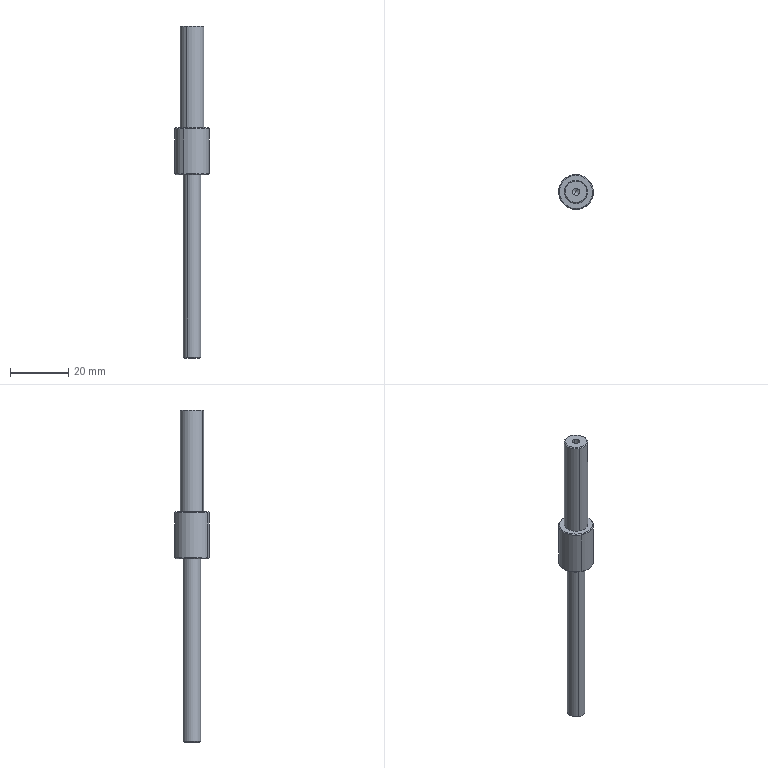Component | SolidWorks | DZ.KX.203-TC1505-20-18-05-96-1 | 1 solid | 26 faces | box 12 x 12 x 114 mm | volume 5230 mm3 | cone 12 | cylinder 10 | plane 4 | commonest cylinder face diameters 2.5 x4 6 x2 12 x2 8 x2 | material Plain Carbon Steel
build123d program:
from build123d import *

# Parameters (mm, degrees)
M3_TAPPED_HOLE1_D     = 2.5
M3_TAPPED_HOLE1_DEPTH = 12.5
M3_TAPPED_HOLE1_TIP   = 0.7511
CHAMFER1_SIZE         = 0.3
M3_TAPPED_HOLE2_D     = 2.5
M3_TAPPED_HOLE2_DEPTH = 10.5
M3_TAPPED_HOLE2_TIP   = 0.7511


with BuildPart() as part:
    # Sketch1 → Revolve1 (revolve)
    with BuildSketch(Plane(origin=(0, 0, 0), x_dir=(0, 0, -1), z_dir=(1, 0, 0))):
        Polygon((0, 0), (0, 114), (4, 114), (4, 79), (6, 79), (6, 63), (3, 63), (3, 0), align=None)
    revolve(axis=Axis((0, 0, 0), (0, 1, 0)))

    # M3 Tapped Hole1
    with Locations(Plane(origin=(0, 114, 0), x_dir=(1, 0, 0), z_dir=(0, 1, 0))):
        with Locations((0, 0)):
            Hole(M3_TAPPED_HOLE1_D / 2, depth=M3_TAPPED_HOLE1_DEPTH)
            with Locations((0, 0, -(M3_TAPPED_HOLE1_DEPTH + M3_TAPPED_HOLE1_TIP / 2))):  # 118° drill point
                Cone(0, M3_TAPPED_HOLE1_D / 2, M3_TAPPED_HOLE1_TIP, mode=Mode.SUBTRACT)

    # Chamfer1
    chamfer1_edges = [part.edges().sort_by_distance(p)[0] for p in [
        (0, 0, 3),
        (0, 63, 6),
        (0, 79, 6),
        (0, 114, 4),
    ]]
    chamfer(chamfer1_edges, length=CHAMFER1_SIZE)

    # M3 Tapped Hole2
    with Locations(Plane(origin=(0, 0, 0), x_dir=(-1, 0, 0), z_dir=(0, -1, 0))):
        with Locations((0, 0)):
            Hole(M3_TAPPED_HOLE2_D / 2, depth=M3_TAPPED_HOLE2_DEPTH)
            with Locations((0, 0, -(M3_TAPPED_HOLE2_DEPTH + M3_TAPPED_HOLE2_TIP / 2))):  # 118° drill point
                Cone(0, M3_TAPPED_HOLE2_D / 2, M3_TAPPED_HOLE2_TIP, mode=Mode.SUBTRACT)


solid = part.part

# Placed as in the assembly
solid = solid.moved(Location((295.5, -817.807, 24.06), (90, 0, 0)))
STEP:
#1=COLOUR_RGB('',0.7922,0.8196,0.9333);
#2=FILL_AREA_STYLE_COLOUR('',#1);
#3=FILL_AREA_STYLE('',(#2));
#4=SURFACE_STYLE_FILL_AREA(#3);
#5=SURFACE_SIDE_STYLE('',(#4));
#6=SURFACE_STYLE_USAGE(.BOTH.,#5);
#7=PRESENTATION_STYLE_ASSIGNMENT((#6));
#8=CARTESIAN_POINT('',(11.61,-32.24,1.361));
#9=VERTEX_POINT('',#8);
#10=CARTESIAN_POINT('',(11.657,-32.154,1.361));
#11=VERTEX_POINT('',#10);
#12=CARTESIAN_POINT('',(11.634,-32.197,1.361));
#13=DIRECTION('',(0.,-0.,-1.));
#14=DIRECTION('',(0.4749,0.88,0.));
#15=AXIS2_PLACEMENT_3D('',#12,#13,#14);
#16=CIRCLE('',#15,0.04921);
#17=EDGE_CURVE('',#9,#11,#16,.T.);
#18=ORIENTED_EDGE('',*,*,#17,.F.);
#19=CARTESIAN_POINT('',(11.61,-32.24,0.9472));
#20=VERTEX_POINT('',#19);
#21=CARTESIAN_POINT('',(11.61,-32.24,0.9472));
#22=DIRECTION('',(0.,-0.,-1.));
#23=VECTOR('',#22,39.37);
#24=LINE('',#21,#23);
#25=EDGE_CURVE('',#9,#20,#24,.T.);
#26=ORIENTED_EDGE('',*,*,#25,.T.);
#27=CARTESIAN_POINT('',(11.657,-32.154,0.9472));
#28=VERTEX_POINT('',#27);
#29=CARTESIAN_POINT('',(11.634,-32.197,0.9472));
#30=DIRECTION('',(0.,-0.,-1.));
#31=DIRECTION('',(0.4749,0.88,-0.));
#32=AXIS2_PLACEMENT_3D('',#29,#30,#31);
#33=CIRCLE('',#32,0.04921);
#34=EDGE_CURVE('',#20,#28,#33,.T.);
#35=ORIENTED_EDGE('',*,*,#34,.T.);
#36=CARTESIAN_POINT('',(11.657,-32.154,0.9472));
#37=DIRECTION('',(0.,-0.,-1.));
#38=VECTOR('',#37,39.37);
#39=LINE('',#36,#38);
#40=EDGE_CURVE('',#11,#28,#39,.T.);
#41=ORIENTED_EDGE('',*,*,#40,.F.);
#42=EDGE_LOOP('',(#18,#26,#35,#41));
#43=FACE_OUTER_BOUND('',#42,.T.);
#44=CARTESIAN_POINT('',(11.634,-32.197,0.9472));
#45=DIRECTION('',(0.,-0.,-1.));
#46=DIRECTION('',(0.4749,0.88,-0.));
#47=AXIS2_PLACEMENT_3D('',#44,#45,#46);
#48=CYLINDRICAL_SURFACE('',#47,0.04921);
#49=ADVANCED_FACE('',(#43),#48,.F.);
#50=CARTESIAN_POINT('',(11.634,-32.197,1.39));
#51=VERTEX_POINT('',#50);
#52=CARTESIAN_POINT('',(11.657,-32.154,1.361));
#53=DIRECTION('',(0.4071,0.7543,-0.515));
#54=VECTOR('',#53,39.37);
#55=LINE('',#52,#54);
#56=EDGE_CURVE('',#51,#11,#55,.T.);
#57=ORIENTED_EDGE('',*,*,#56,.F.);
#58=CARTESIAN_POINT('',(11.61,-32.24,1.361));
#59=DIRECTION('',(-0.4071,-0.7543,-0.515));
#60=VECTOR('',#59,39.37);
#61=LINE('',#58,#60);
#62=EDGE_CURVE('',#51,#9,#61,.T.);
#63=ORIENTED_EDGE('',*,*,#62,.T.);
#64=ORIENTED_EDGE('',*,*,#17,.T.);
#65=EDGE_LOOP('',(#57,#63,#64));
#66=FACE_OUTER_BOUND('',#65,.T.);
#67=CARTESIAN_POINT('',(11.634,-32.197,1.361));
#68=DIRECTION('',(0.,-0.,-1.));
#69=DIRECTION('',(0.4749,0.88,0.));
#70=AXIS2_PLACEMENT_3D('',#67,#68,#69);
#71=CONICAL_SURFACE('',#70,0.04921,1.03);
#72=ADVANCED_FACE('',(#66),#71,.F.);
#73=CARTESIAN_POINT('',(11.565,-32.325,5.435));
#74=VERTEX_POINT('',#73);
#75=CARTESIAN_POINT('',(11.703,-32.069,5.435));
#76=VERTEX_POINT('',#75);
#77=CARTESIAN_POINT('',(11.634,-32.197,5.435));
#78=DIRECTION('',(-0.,0.,1.));
#79=DIRECTION('',(-0.4749,-0.88,0.));
#80=AXIS2_PLACEMENT_3D('',#77,#78,#79);
#81=CIRCLE('',#80,0.1457);
#82=EDGE_CURVE('',#74,#76,#81,.T.);
#83=ORIENTED_EDGE('',*,*,#82,.F.);
#84=CARTESIAN_POINT('',(11.559,-32.336,5.424));
#85=VERTEX_POINT('',#84);
#86=CARTESIAN_POINT('',(11.559,-32.336,5.424));
#87=DIRECTION('',(-0.3358,-0.6223,-0.7071));
#88=VECTOR('',#87,39.37);
#89=LINE('',#86,#88);
#90=EDGE_CURVE('',#74,#85,#89,.T.);
#91=ORIENTED_EDGE('',*,*,#90,.T.);
#92=CARTESIAN_POINT('',(11.709,-32.059,5.424));
#93=VERTEX_POINT('',#92);
#94=CARTESIAN_POINT('',(11.634,-32.197,5.424));
#95=DIRECTION('',(0.,-0.,-1.));
#96=DIRECTION('',(-0.4749,-0.88,0.));
#97=AXIS2_PLACEMENT_3D('',#94,#95,#96);
#98=CIRCLE('',#97,0.1575);
#99=EDGE_CURVE('',#93,#85,#98,.T.);
#100=ORIENTED_EDGE('',*,*,#99,.F.);
#101=CARTESIAN_POINT('',(11.709,-32.059,5.424));
#102=DIRECTION('',(0.3358,0.6223,-0.7071));
#103=VECTOR('',#102,39.37);
#104=LINE('',#101,#103);
#105=EDGE_CURVE('',#76,#93,#104,.T.);
#106=ORIENTED_EDGE('',*,*,#105,.F.);
#107=EDGE_LOOP('',(#83,#91,#100,#106));
#108=FACE_OUTER_BOUND('',#107,.T.);
#109=CARTESIAN_POINT('',(11.634,-32.197,5.424));
#110=DIRECTION('',(0.,-0.,-1.));
#111=DIRECTION('',(0.4749,0.88,0.));
#112=AXIS2_PLACEMENT_3D('',#109,#110,#111);
#113=CONICAL_SURFACE('',#112,0.1575,0.7854);
#114=ADVANCED_FACE('',(#108),#113,.T.);
#115=CARTESIAN_POINT('',(11.684,-32.104,0.9472));
#116=VERTEX_POINT('',#115);
#117=CARTESIAN_POINT('',(11.583,-32.291,0.9472));
#118=VERTEX_POINT('',#117);
#119=CARTESIAN_POINT('',(11.634,-32.197,0.9472));
#120=DIRECTION('',(0.,-0.,-1.));
#121=DIRECTION('',(0.4749,0.88,-0.));
#122=AXIS2_PLACEMENT_3D('',#119,#120,#121);
#123=CIRCLE('',#122,0.1063);
#124=EDGE_CURVE('',#116,#118,#123,.T.);
#125=ORIENTED_EDGE('',*,*,#124,.F.);
#126=CARTESIAN_POINT('',(11.69,-32.093,0.959));
#127=VERTEX_POINT('',#126);
#128=CARTESIAN_POINT('',(11.684,-32.104,0.9472));
#129=DIRECTION('',(0.3358,0.6223,0.7071));
#130=VECTOR('',#129,39.37);
#131=LINE('',#128,#130);
#132=EDGE_CURVE('',#116,#127,#131,.T.);
#133=ORIENTED_EDGE('',*,*,#132,.T.);
#134=CARTESIAN_POINT('',(11.578,-32.301,0.959));
#135=VERTEX_POINT('',#134);
#136=CARTESIAN_POINT('',(11.634,-32.197,0.959));
#137=DIRECTION('',(-0.,0.,1.));
#138=DIRECTION('',(0.4749,0.88,-0.));
#139=AXIS2_PLACEMENT_3D('',#136,#137,#138);
#140=CIRCLE('',#139,0.1181);
#141=EDGE_CURVE('',#135,#127,#140,.T.);
#142=ORIENTED_EDGE('',*,*,#141,.F.);
#143=CARTESIAN_POINT('',(11.583,-32.291,0.9472));
#144=DIRECTION('',(-0.3358,-0.6223,0.7071));
#145=VECTOR('',#144,39.37);
#146=LINE('',#143,#145);
#147=EDGE_CURVE('',#118,#135,#146,.T.);
#148=ORIENTED_EDGE('',*,*,#147,.F.);
#149=EDGE_LOOP('',(#125,#133,#142,#148));
#150=FACE_OUTER_BOUND('',#149,.T.);
#151=CARTESIAN_POINT('',(11.634,-32.197,0.9472));
#152=DIRECTION('',(-0.,0.,1.));
#153=DIRECTION('',(-0.4749,-0.88,0.));
#154=AXIS2_PLACEMENT_3D('',#151,#152,#153);
#155=CONICAL_SURFACE('',#154,0.1063,0.7854);
#156=ADVANCED_FACE('',(#150),#155,.T.);
#157=CARTESIAN_POINT('',(11.527,-32.395,4.057));
#158=VERTEX_POINT('',#157);
#159=CARTESIAN_POINT('',(11.74,-32.,4.057));
#160=VERTEX_POINT('',#159);
#161=CARTESIAN_POINT('',(11.634,-32.197,4.057));
#162=DIRECTION('',(-0.,0.,1.));
#163=DIRECTION('',(-0.4749,-0.88,0.));
#164=AXIS2_PLACEMENT_3D('',#161,#162,#163);
#165=CIRCLE('',#164,0.2244);
#166=EDGE_CURVE('',#158,#160,#165,.T.);
#167=ORIENTED_EDGE('',*,*,#166,.F.);
#168=CARTESIAN_POINT('',(11.522,-32.405,4.046));
#169=VERTEX_POINT('',#168);
#170=CARTESIAN_POINT('',(11.522,-32.405,4.046));
#171=DIRECTION('',(-0.3358,-0.6223,-0.7071));
#172=VECTOR('',#171,39.37);
#173=LINE('',#170,#172);
#174=EDGE_CURVE('',#158,#169,#173,.T.);
#175=ORIENTED_EDGE('',*,*,#174,.T.);
#176=CARTESIAN_POINT('',(11.746,-31.989,4.046));
#177=VERTEX_POINT('',#176);
#178=CARTESIAN_POINT('',(11.634,-32.197,4.046));
#179=DIRECTION('',(0.,-0.,-1.));
#180=DIRECTION('',(-0.4749,-0.88,0.));
#181=AXIS2_PLACEMENT_3D('',#178,#179,#180);
#182=CIRCLE('',#181,0.2362);
#183=EDGE_CURVE('',#177,#169,#182,.T.);
#184=ORIENTED_EDGE('',*,*,#183,.F.);
#185=CARTESIAN_POINT('',(11.746,-31.989,4.046));
#186=DIRECTION('',(0.3358,0.6223,-0.7071));
#187=VECTOR('',#186,39.37);
#188=LINE('',#185,#187);
#189=EDGE_CURVE('',#160,#177,#188,.T.);
#190=ORIENTED_EDGE('',*,*,#189,.F.);
#191=EDGE_LOOP('',(#167,#175,#184,#190));
#192=FACE_OUTER_BOUND('',#191,.T.);
#193=CARTESIAN_POINT('',(11.634,-32.197,4.046));
#194=DIRECTION('',(0.,-0.,-1.));
#195=DIRECTION('',(0.4749,0.88,-0.));
#196=AXIS2_PLACEMENT_3D('',#193,#194,#195);
#197=CONICAL_SURFACE('',#196,0.2362,0.7854);
#198=ADVANCED_FACE('',(#192),#197,.T.);
#199=CARTESIAN_POINT('',(11.74,-32.,3.428));
#200=VERTEX_POINT('',#199);
#201=CARTESIAN_POINT('',(11.527,-32.395,3.428));
#202=VERTEX_POINT('',#201);
#203=CARTESIAN_POINT('',(11.634,-32.197,3.428));
#204=DIRECTION('',(0.,-0.,-1.));
#205=DIRECTION('',(0.4749,0.88,-0.));
#206=AXIS2_PLACEMENT_3D('',#203,#204,#205);
#207=CIRCLE('',#206,0.2244);
#208=EDGE_CURVE('',#200,#202,#207,.T.);
#209=ORIENTED_EDGE('',*,*,#208,.F.);
#210=CARTESIAN_POINT('',(11.746,-31.989,3.439));
#211=VERTEX_POINT('',#210);
#212=CARTESIAN_POINT('',(11.74,-32.,3.428));
#213=DIRECTION('',(0.3358,0.6223,0.7071));
#214=VECTOR('',#213,39.37);
#215=LINE('',#212,#214);
#216=EDGE_CURVE('',#200,#211,#215,.T.);
#217=ORIENTED_EDGE('',*,*,#216,.T.);
#218=CARTESIAN_POINT('',(11.522,-32.405,3.439));
#219=VERTEX_POINT('',#218);
#220=CARTESIAN_POINT('',(11.634,-32.197,3.439));
#221=DIRECTION('',(-0.,0.,1.));
#222=DIRECTION('',(0.4749,0.88,-0.));
#223=AXIS2_PLACEMENT_3D('',#220,#221,#222);
#224=CIRCLE('',#223,0.2362);
#225=EDGE_CURVE('',#219,#211,#224,.T.);
#226=ORIENTED_EDGE('',*,*,#225,.F.);
#227=CARTESIAN_POINT('',(11.527,-32.395,3.428));
#228=DIRECTION('',(-0.3358,-0.6223,0.7071));
#229=VECTOR('',#228,39.37);
#230=LINE('',#227,#229);
#231=EDGE_CURVE('',#202,#219,#230,.T.);
#232=ORIENTED_EDGE('',*,*,#231,.F.);
#233=EDGE_LOOP('',(#209,#217,#226,#232));
#234=FACE_OUTER_BOUND('',#233,.T.);
#235=CARTESIAN_POINT('',(11.634,-32.197,3.428));
#236=DIRECTION('',(-0.,0.,1.));
#237=DIRECTION('',(-0.4749,-0.88,0.));
#238=AXIS2_PLACEMENT_3D('',#235,#236,#237);
#239=CONICAL_SURFACE('',#238,0.2244,0.7854);
#240=ADVANCED_FACE('',(#234),#239,.T.);
#241=CARTESIAN_POINT('',(11.657,-32.154,4.943));
#242=VERTEX_POINT('',#241);
#243=CARTESIAN_POINT('',(11.61,-32.24,4.943));
#244=VERTEX_POINT('',#243);
#245=CARTESIAN_POINT('',(11.634,-32.197,4.943));
#246=DIRECTION('',(-0.,0.,1.));
#247=DIRECTION('',(-0.4749,-0.88,0.));
#248=AXIS2_PLACEMENT_3D('',#245,#246,#247);
#249=CIRCLE('',#248,0.04921);
#250=EDGE_CURVE('',#242,#244,#249,.T.);
#251=ORIENTED_EDGE('',*,*,#250,.F.);
#252=CARTESIAN_POINT('',(11.657,-32.154,5.435));
#253=VERTEX_POINT('',#252);
#254=CARTESIAN_POINT('',(11.657,-32.154,5.435));
#255=DIRECTION('',(-0.,0.,1.));
#256=VECTOR('',#255,39.37);
#257=LINE('',#254,#256);
#258=EDGE_CURVE('',#242,#253,#257,.T.);
#259=ORIENTED_EDGE('',*,*,#258,.T.);
#260=CARTESIAN_POINT('',(11.61,-32.24,5.435));
#261=VERTEX_POINT('',#260);
#262=CARTESIAN_POINT('',(11.634,-32.197,5.435));
#263=DIRECTION('',(-0.,0.,1.));
#264=DIRECTION('',(-0.4749,-0.88,0.));
#265=AXIS2_PLACEMENT_3D('',#262,#263,#264);
#266=CIRCLE('',#265,0.04921);
#267=EDGE_CURVE('',#253,#261,#266,.T.);
#268=ORIENTED_EDGE('',*,*,#267,.T.);
#269=CARTESIAN_POINT('',(11.61,-32.24,5.435));
#270=DIRECTION('',(-0.,0.,1.));
#271=VECTOR('',#270,39.37);
#272=LINE('',#269,#271);
#273=EDGE_CURVE('',#244,#261,#272,.T.);
#274=ORIENTED_EDGE('',*,*,#273,.F.);
#275=EDGE_LOOP('',(#251,#259,#268,#274));
#276=FACE_OUTER_BOUND('',#275,.T.);
#277=CARTESIAN_POINT('',(11.634,-32.197,5.435));
#278=DIRECTION('',(-0.,0.,1.));
#279=DIRECTION('',(-0.4749,-0.88,0.));
#280=AXIS2_PLACEMENT_3D('',#277,#278,#279);
#281=CYLINDRICAL_SURFACE('',#280,0.04921);
#282=ADVANCED_FACE('',(#276),#281,.F.);
#283=CARTESIAN_POINT('',(11.634,-32.197,4.914));
#284=VERTEX_POINT('',#283);
#285=CARTESIAN_POINT('',(11.61,-32.24,4.943));
#286=DIRECTION('',(-0.4071,-0.7543,0.515));
#287=VECTOR('',#286,39.37);
#288=LINE('',#285,#287);
#289=EDGE_CURVE('',#284,#244,#288,.T.);
#290=ORIENTED_EDGE('',*,*,#289,.F.);
#291=CARTESIAN_POINT('',(11.657,-32.154,4.943));
#292=DIRECTION('',(0.4071,0.7543,0.515));
#293=VECTOR('',#292,39.37);
#294=LINE('',#291,#293);
#295=EDGE_CURVE('',#284,#242,#294,.T.);
#296=ORIENTED_EDGE('',*,*,#295,.T.);
#297=ORIENTED_EDGE('',*,*,#250,.T.);
#298=EDGE_LOOP('',(#290,#296,#297));
#299=FACE_OUTER_BOUND('',#298,.T.);
#300=CARTESIAN_POINT('',(11.634,-32.197,4.943));
#301=DIRECTION('',(-0.,0.,1.));
#302=DIRECTION('',(-0.4749,-0.88,0.));
#303=AXIS2_PLACEMENT_3D('',#300,#301,#302);
#304=CONICAL_SURFACE('',#303,0.04921,1.03);
#305=ADVANCED_FACE('',(#299),#304,.F.);
#306=CARTESIAN_POINT('',(11.69,-32.093,3.428));
#307=VERTEX_POINT('',#306);
#308=CARTESIAN_POINT('',(11.578,-32.301,3.428));
#309=VERTEX_POINT('',#308);
#310=CARTESIAN_POINT('',(11.634,-32.197,3.428));
#311=DIRECTION('',(0.,-0.,-1.));
#312=DIRECTION('',(0.4749,0.88,-0.));
#313=AXIS2_PLACEMENT_3D('',#310,#311,#312);
#314=CIRCLE('',#313,0.1181);
#315=EDGE_CURVE('',#307,#309,#314,.T.);
#316=ORIENTED_EDGE('',*,*,#315,.T.);
#317=CARTESIAN_POINT('',(11.578,-32.301,0.9472));
#318=DIRECTION('',(0.,-0.,-1.));
#319=VECTOR('',#318,39.37);
#320=LINE('',#317,#319);
#321=EDGE_CURVE('',#309,#135,#320,.T.);
#322=ORIENTED_EDGE('',*,*,#321,.T.);
#323=ORIENTED_EDGE('',*,*,#141,.T.);
#324=CARTESIAN_POINT('',(11.69,-32.093,0.9472));
#325=DIRECTION('',(0.,-0.,-1.));
#326=VECTOR('',#325,39.37);
#327=LINE('',#324,#326);
#328=EDGE_CURVE('',#307,#127,#327,.T.);
#329=ORIENTED_EDGE('',*,*,#328,.F.);
#330=EDGE_LOOP('',(#316,#322,#323,#329));
#331=FACE_OUTER_BOUND('',#330,.T.);
#332=CARTESIAN_POINT('',(11.634,-32.197,0.9472));
#333=DIRECTION('',(0.,-0.,-1.));
#334=DIRECTION('',(0.4749,0.88,-0.));
#335=AXIS2_PLACEMENT_3D('',#332,#333,#334);
#336=CYLINDRICAL_SURFACE('',#335,0.1181);
#337=ADVANCED_FACE('',(#331),#336,.T.);
#338=ORIENTED_EDGE('',*,*,#183,.T.);
#339=CARTESIAN_POINT('',(11.522,-32.405,0.9472));
#340=DIRECTION('',(0.,-0.,-1.));
#341=VECTOR('',#340,39.37);
#342=LINE('',#339,#341);
#343=EDGE_CURVE('',#169,#219,#342,.T.);
#344=ORIENTED_EDGE('',*,*,#343,.T.);
#345=ORIENTED_EDGE('',*,*,#225,.T.);
#346=CARTESIAN_POINT('',(11.746,-31.989,0.9472));
#347=DIRECTION('',(0.,-0.,-1.));
#348=VECTOR('',#347,39.37);
#349=LINE('',#346,#348);
#350=EDGE_CURVE('',#177,#211,#349,.T.);
#351=ORIENTED_EDGE('',*,*,#350,.F.);
#352=EDGE_LOOP('',(#338,#344,#345,#351));
#353=FACE_OUTER_BOUND('',#352,.T.);
#354=CARTESIAN_POINT('',(11.634,-32.197,0.9472));
#355=DIRECTION('',(0.,-0.,-1.));
#356=DIRECTION('',(0.4749,0.88,-0.));
#357=AXIS2_PLACEMENT_3D('',#354,#355,#356);
#358=CYLINDRICAL_SURFACE('',#357,0.2362);
#359=ADVANCED_FACE('',(#353),#358,.T.);
#360=ORIENTED_EDGE('',*,*,#99,.T.);
#361=CARTESIAN_POINT('',(11.559,-32.336,4.057));
#362=VERTEX_POINT('',#361);
#363=CARTESIAN_POINT('',(11.559,-32.336,0.9472));
#364=DIRECTION('',(0.,-0.,-1.));
#365=VECTOR('',#364,39.37);
#366=LINE('',#363,#365);
#367=EDGE_CURVE('',#85,#362,#366,.T.);
#368=ORIENTED_EDGE('',*,*,#367,.T.);
#369=CARTESIAN_POINT('',(11.709,-32.059,4.057));
#370=VERTEX_POINT('',#369);
#371=CARTESIAN_POINT('',(11.634,-32.197,4.057));
#372=DIRECTION('',(0.,-0.,-1.));
#373=DIRECTION('',(0.4749,0.88,-0.));
#374=AXIS2_PLACEMENT_3D('',#371,#372,#373);
#375=CIRCLE('',#374,0.1575);
#376=EDGE_CURVE('',#370,#362,#375,.T.);
#377=ORIENTED_EDGE('',*,*,#376,.F.);
#378=CARTESIAN_POINT('',(11.709,-32.059,0.9472));
#379=DIRECTION('',(0.,-0.,-1.));
#380=VECTOR('',#379,39.37);
#381=LINE('',#378,#380);
#382=EDGE_CURVE('',#93,#370,#381,.T.);
#383=ORIENTED_EDGE('',*,*,#382,.F.);
#384=EDGE_LOOP('',(#360,#368,#377,#383));
#385=FACE_OUTER_BOUND('',#384,.T.);
#386=CARTESIAN_POINT('',(11.634,-32.197,0.9472));
#387=DIRECTION('',(0.,-0.,-1.));
#388=DIRECTION('',(0.4749,0.88,-0.));
#389=AXIS2_PLACEMENT_3D('',#386,#387,#388);
#390=CYLINDRICAL_SURFACE('',#389,0.1575);
#391=ADVANCED_FACE('',(#385),#390,.T.);
#392=CARTESIAN_POINT('',(11.634,-32.197,0.9472));
#393=DIRECTION('',(0.,-0.,-1.));
#394=DIRECTION('',(0.4749,0.88,-0.));
#395=AXIS2_PLACEMENT_3D('',#392,#393,#394);
#396=CIRCLE('',#395,0.04921);
#397=EDGE_CURVE('',#28,#20,#396,.T.);
#398=ORIENTED_EDGE('',*,*,#397,.F.);
#399=ORIENTED_EDGE('',*,*,#34,.F.);
#400=EDGE_LOOP('',(#398,#399));
#401=FACE_BOUND('',#400,.T.);
#402=CARTESIAN_POINT('',(11.634,-32.197,0.9472));
#403=DIRECTION('',(0.,-0.,-1.));
#404=DIRECTION('',(0.4749,0.88,-0.));
#405=AXIS2_PLACEMENT_3D('',#402,#403,#404);
#406=CIRCLE('',#405,0.1063);
#407=EDGE_CURVE('',#118,#116,#406,.T.);
#408=ORIENTED_EDGE('',*,*,#407,.T.);
#409=ORIENTED_EDGE('',*,*,#124,.T.);
#410=EDGE_LOOP('',(#408,#409));
#411=FACE_OUTER_BOUND('',#410,.T.);
#412=CARTESIAN_POINT('',(11.69,-32.093,0.9472));
#413=DIRECTION('',(0.,-0.,-1.));
#414=DIRECTION('',(0.4749,0.88,-0.));
#415=AXIS2_PLACEMENT_3D('',#412,#413,#414);
#416=PLANE('',#415);
#417=ADVANCED_FACE('',(#401,#411),#416,.T.);
#418=CARTESIAN_POINT('',(11.634,-32.197,5.435));
#419=DIRECTION('',(-0.,0.,1.));
#420=DIRECTION('',(-0.4749,-0.88,0.));
#421=AXIS2_PLACEMENT_3D('',#418,#419,#420);
#422=CIRCLE('',#421,0.1457);
#423=EDGE_CURVE('',#76,#74,#422,.T.);
#424=ORIENTED_EDGE('',*,*,#423,.T.);
#425=ORIENTED_EDGE('',*,*,#82,.T.);
#426=EDGE_LOOP('',(#424,#425));
#427=FACE_OUTER_BOUND('',#426,.T.);
#428=CARTESIAN_POINT('',(11.634,-32.197,5.435));
#429=DIRECTION('',(-0.,0.,1.));
#430=DIRECTION('',(-0.4749,-0.88,0.));
#431=AXIS2_PLACEMENT_3D('',#428,#429,#430);
#432=CIRCLE('',#431,0.04921);
#433=EDGE_CURVE('',#261,#253,#432,.T.);
#434=ORIENTED_EDGE('',*,*,#433,.F.);
#435=ORIENTED_EDGE('',*,*,#267,.F.);
#436=EDGE_LOOP('',(#434,#435));
#437=FACE_BOUND('',#436,.T.);
#438=CARTESIAN_POINT('',(11.634,-32.197,5.435));
#439=DIRECTION('',(-0.,0.,1.));
#440=DIRECTION('',(-0.4749,-0.88,0.));
#441=AXIS2_PLACEMENT_3D('',#438,#439,#440);
#442=PLANE('',#441);
#443=ADVANCED_FACE('',(#427,#437),#442,.T.);
#444=ORIENTED_EDGE('',*,*,#367,.F.);
#445=CARTESIAN_POINT('',(11.634,-32.197,5.424));
#446=DIRECTION('',(0.,-0.,-1.));
#447=DIRECTION('',(-0.4749,-0.88,0.));
#448=AXIS2_PLACEMENT_3D('',#445,#446,#447);
#449=CIRCLE('',#448,0.1575);
#450=EDGE_CURVE('',#85,#93,#449,.T.);
#451=ORIENTED_EDGE('',*,*,#450,.T.);
#452=ORIENTED_EDGE('',*,*,#382,.T.);
#453=CARTESIAN_POINT('',(11.634,-32.197,4.057));
#454=DIRECTION('',(0.,-0.,-1.));
#455=DIRECTION('',(0.4749,0.88,-0.));
#456=AXIS2_PLACEMENT_3D('',#453,#454,#455);
#457=CIRCLE('',#456,0.1575);
#458=EDGE_CURVE('',#362,#370,#457,.T.);
#459=ORIENTED_EDGE('',*,*,#458,.F.);
#460=EDGE_LOOP('',(#444,#451,#452,#459));
#461=FACE_OUTER_BOUND('',#460,.T.);
#462=CARTESIAN_POINT('',(11.634,-32.197,0.9472));
#463=DIRECTION('',(0.,-0.,-1.));
#464=DIRECTION('',(0.4749,0.88,-0.));
#465=AXIS2_PLACEMENT_3D('',#462,#463,#464);
#466=CYLINDRICAL_SURFACE('',#465,0.1575);
#467=ADVANCED_FACE('',(#461),#466,.T.);
#468=CARTESIAN_POINT('',(11.634,-32.197,4.057));
#469=DIRECTION('',(-0.,0.,1.));
#470=DIRECTION('',(-0.4749,-0.88,0.));
#471=AXIS2_PLACEMENT_3D('',#468,#469,#470);
#472=CIRCLE('',#471,0.2244);
#473=EDGE_CURVE('',#160,#158,#472,.T.);
#474=ORIENTED_EDGE('',*,*,#473,.T.);
#475=ORIENTED_EDGE('',*,*,#166,.T.);
#476=EDGE_LOOP('',(#474,#475));
#477=FACE_OUTER_BOUND('',#476,.T.);
#478=ORIENTED_EDGE('',*,*,#376,.T.);
#479=ORIENTED_EDGE('',*,*,#458,.T.);
#480=EDGE_LOOP('',(#478,#479));
#481=FACE_BOUND('',#480,.T.);
#482=CARTESIAN_POINT('',(11.709,-32.059,4.057));
#483=DIRECTION('',(-0.,0.,1.));
#484=DIRECTION('',(-0.4749,-0.88,0.));
#485=AXIS2_PLACEMENT_3D('',#482,#483,#484);
#486=PLANE('',#485);
#487=ADVANCED_FACE('',(#477,#481),#486,.T.);
#488=ORIENTED_EDGE('',*,*,#343,.F.);
#489=CARTESIAN_POINT('',(11.634,-32.197,4.046));
#490=DIRECTION('',(0.,-0.,-1.));
#491=DIRECTION('',(-0.4749,-0.88,0.));
#492=AXIS2_PLACEMENT_3D('',#489,#490,#491);
#493=CIRCLE('',#492,0.2362);
#494=EDGE_CURVE('',#169,#177,#493,.T.);
#495=ORIENTED_EDGE('',*,*,#494,.T.);
#496=ORIENTED_EDGE('',*,*,#350,.T.);
#497=CARTESIAN_POINT('',(11.634,-32.197,3.439));
#498=DIRECTION('',(-0.,0.,1.));
#499=DIRECTION('',(0.4749,0.88,-0.));
#500=AXIS2_PLACEMENT_3D('',#497,#498,#499);
#501=CIRCLE('',#500,0.2362);
#502=EDGE_CURVE('',#211,#219,#501,.T.);
#503=ORIENTED_EDGE('',*,*,#502,.T.);
#504=EDGE_LOOP('',(#488,#495,#496,#503));
#505=FACE_OUTER_BOUND('',#504,.T.);
#506=CARTESIAN_POINT('',(11.634,-32.197,0.9472));
#507=DIRECTION('',(0.,-0.,-1.));
#508=DIRECTION('',(0.4749,0.88,-0.));
#509=AXIS2_PLACEMENT_3D('',#506,#507,#508);
#510=CYLINDRICAL_SURFACE('',#509,0.2362);
#511=ADVANCED_FACE('',(#505),#510,.T.);
#512=CARTESIAN_POINT('',(11.634,-32.197,3.428));
#513=DIRECTION('',(0.,-0.,-1.));
#514=DIRECTION('',(0.4749,0.88,-0.));
#515=AXIS2_PLACEMENT_3D('',#512,#513,#514);
#516=CIRCLE('',#515,0.2244);
#517=EDGE_CURVE('',#202,#200,#516,.T.);
#518=ORIENTED_EDGE('',*,*,#517,.T.);
#519=ORIENTED_EDGE('',*,*,#208,.T.);
#520=EDGE_LOOP('',(#518,#519));
#521=FACE_OUTER_BOUND('',#520,.T.);
#522=ORIENTED_EDGE('',*,*,#315,.F.);
#523=CARTESIAN_POINT('',(11.634,-32.197,3.428));
#524=DIRECTION('',(0.,-0.,-1.));
#525=DIRECTION('',(0.4749,0.88,-0.));
#526=AXIS2_PLACEMENT_3D('',#523,#524,#525);
#527=CIRCLE('',#526,0.1181);
#528=EDGE_CURVE('',#309,#307,#527,.T.);
#529=ORIENTED_EDGE('',*,*,#528,.F.);
#530=EDGE_LOOP('',(#522,#529));
#531=FACE_BOUND('',#530,.T.);
#532=CARTESIAN_POINT('',(11.746,-31.989,3.428));
#533=DIRECTION('',(0.,-0.,-1.));
#534=DIRECTION('',(0.4749,0.88,-0.));
#535=AXIS2_PLACEMENT_3D('',#532,#533,#534);
#536=PLANE('',#535);
#537=ADVANCED_FACE('',(#521,#531),#536,.T.);
#538=ORIENTED_EDGE('',*,*,#321,.F.);
#539=ORIENTED_EDGE('',*,*,#528,.T.);
#540=ORIENTED_EDGE('',*,*,#328,.T.);
#541=CARTESIAN_POINT('',(11.634,-32.197,0.959));
#542=DIRECTION('',(-0.,0.,1.));
#543=DIRECTION('',(0.4749,0.88,-0.));
#544=AXIS2_PLACEMENT_3D('',#541,#542,#543);
#545=CIRCLE('',#544,0.1181);
#546=EDGE_CURVE('',#127,#135,#545,.T.);
#547=ORIENTED_EDGE('',*,*,#546,.T.);
#548=EDGE_LOOP('',(#538,#539,#540,#547));
#549=FACE_OUTER_BOUND('',#548,.T.);
#550=CARTESIAN_POINT('',(11.634,-32.197,0.9472));
#551=DIRECTION('',(0.,-0.,-1.));
#552=DIRECTION('',(0.4749,0.88,-0.));
#553=AXIS2_PLACEMENT_3D('',#550,#551,#552);
#554=CYLINDRICAL_SURFACE('',#553,0.1181);
#555=ADVANCED_FACE('',(#549),#554,.T.);
#556=ORIENTED_EDGE('',*,*,#295,.F.);
#557=ORIENTED_EDGE('',*,*,#289,.T.);
#558=CARTESIAN_POINT('',(11.634,-32.197,4.943));
#559=DIRECTION('',(-0.,0.,1.));
#560=DIRECTION('',(-0.4749,-0.88,0.));
#561=AXIS2_PLACEMENT_3D('',#558,#559,#560);
#562=CIRCLE('',#561,0.04921);
#563=EDGE_CURVE('',#244,#242,#562,.T.);
#564=ORIENTED_EDGE('',*,*,#563,.T.);
#565=EDGE_LOOP('',(#556,#557,#564));
#566=FACE_OUTER_BOUND('',#565,.T.);
#567=CARTESIAN_POINT('',(11.634,-32.197,4.943));
#568=DIRECTION('',(-0.,0.,1.));
#569=DIRECTION('',(-0.4749,-0.88,0.));
#570=AXIS2_PLACEMENT_3D('',#567,#568,#569);
#571=CONICAL_SURFACE('',#570,0.04921,1.03);
#572=ADVANCED_FACE('',(#566),#571,.F.);
#573=ORIENTED_EDGE('',*,*,#258,.F.);
#574=ORIENTED_EDGE('',*,*,#563,.F.);
#575=ORIENTED_EDGE('',*,*,#273,.T.);
#576=ORIENTED_EDGE('',*,*,#433,.T.);
#577=EDGE_LOOP('',(#573,#574,#575,#576));
#578=FACE_OUTER_BOUND('',#577,.T.);
#579=CARTESIAN_POINT('',(11.634,-32.197,5.435));
#580=DIRECTION('',(-0.,0.,1.));
#581=DIRECTION('',(-0.4749,-0.88,0.));
#582=AXIS2_PLACEMENT_3D('',#579,#580,#581);
#583=CYLINDRICAL_SURFACE('',#582,0.04921);
#584=ADVANCED_FACE('',(#578),#583,.F.);
#585=ORIENTED_EDGE('',*,*,#216,.F.);
#586=ORIENTED_EDGE('',*,*,#517,.F.);
#587=ORIENTED_EDGE('',*,*,#231,.T.);
#588=ORIENTED_EDGE('',*,*,#502,.F.);
#589=EDGE_LOOP('',(#585,#586,#587,#588));
#590=FACE_OUTER_BOUND('',#589,.T.);
#591=CARTESIAN_POINT('',(11.634,-32.197,3.428));
#592=DIRECTION('',(-0.,0.,1.));
#593=DIRECTION('',(-0.4749,-0.88,0.));
#594=AXIS2_PLACEMENT_3D('',#591,#592,#593);
#595=CONICAL_SURFACE('',#594,0.2244,0.7854);
#596=ADVANCED_FACE('',(#590),#595,.T.);
#597=ORIENTED_EDGE('',*,*,#174,.F.);
#598=ORIENTED_EDGE('',*,*,#473,.F.);
#599=ORIENTED_EDGE('',*,*,#189,.T.);
#600=ORIENTED_EDGE('',*,*,#494,.F.);
#601=EDGE_LOOP('',(#597,#598,#599,#600));
#602=FACE_OUTER_BOUND('',#601,.T.);
#603=CARTESIAN_POINT('',(11.634,-32.197,4.046));
#604=DIRECTION('',(0.,-0.,-1.));
#605=DIRECTION('',(0.4749,0.88,-0.));
#606=AXIS2_PLACEMENT_3D('',#603,#604,#605);
#607=CONICAL_SURFACE('',#606,0.2362,0.7854);
#608=ADVANCED_FACE('',(#602),#607,.T.);
#609=ORIENTED_EDGE('',*,*,#132,.F.);
#610=ORIENTED_EDGE('',*,*,#407,.F.);
#611=ORIENTED_EDGE('',*,*,#147,.T.);
#612=ORIENTED_EDGE('',*,*,#546,.F.);
#613=EDGE_LOOP('',(#609,#610,#611,#612));
#614=FACE_OUTER_BOUND('',#613,.T.);
#615=CARTESIAN_POINT('',(11.634,-32.197,0.9472));
#616=DIRECTION('',(-0.,0.,1.));
#617=DIRECTION('',(-0.4749,-0.88,0.));
#618=AXIS2_PLACEMENT_3D('',#615,#616,#617);
#619=CONICAL_SURFACE('',#618,0.1063,0.7854);
#620=ADVANCED_FACE('',(#614),#619,.T.);
#621=ORIENTED_EDGE('',*,*,#90,.F.);
#622=ORIENTED_EDGE('',*,*,#423,.F.);
#623=ORIENTED_EDGE('',*,*,#105,.T.);
#624=ORIENTED_EDGE('',*,*,#450,.F.);
#625=EDGE_LOOP('',(#621,#622,#623,#624));
#626=FACE_OUTER_BOUND('',#625,.T.);
#627=CARTESIAN_POINT('',(11.634,-32.197,5.424));
#628=DIRECTION('',(0.,-0.,-1.));
#629=DIRECTION('',(0.4749,0.88,0.));
#630=AXIS2_PLACEMENT_3D('',#627,#628,#629);
#631=CONICAL_SURFACE('',#630,0.1575,0.7854);
#632=ADVANCED_FACE('',(#626),#631,.T.);
#633=ORIENTED_EDGE('',*,*,#62,.F.);
#634=ORIENTED_EDGE('',*,*,#56,.T.);
#635=CARTESIAN_POINT('',(11.634,-32.197,1.361));
#636=DIRECTION('',(0.,-0.,-1.));
#637=DIRECTION('',(0.4749,0.88,0.));
#638=AXIS2_PLACEMENT_3D('',#635,#636,#637);
#639=CIRCLE('',#638,0.04921);
#640=EDGE_CURVE('',#11,#9,#639,.T.);
#641=ORIENTED_EDGE('',*,*,#640,.T.);
#642=EDGE_LOOP('',(#633,#634,#641));
#643=FACE_OUTER_BOUND('',#642,.T.);
#644=CARTESIAN_POINT('',(11.634,-32.197,1.361));
#645=DIRECTION('',(0.,-0.,-1.));
#646=DIRECTION('',(0.4749,0.88,0.));
#647=AXIS2_PLACEMENT_3D('',#644,#645,#646);
#648=CONICAL_SURFACE('',#647,0.04921,1.03);
#649=ADVANCED_FACE('',(#643),#648,.F.);
#650=ORIENTED_EDGE('',*,*,#25,.F.);
#651=ORIENTED_EDGE('',*,*,#640,.F.);
#652=ORIENTED_EDGE('',*,*,#40,.T.);
#653=ORIENTED_EDGE('',*,*,#397,.T.);
#654=EDGE_LOOP('',(#650,#651,#652,#653));
#655=FACE_OUTER_BOUND('',#654,.T.);
#656=CARTESIAN_POINT('',(11.634,-32.197,0.9472));
#657=DIRECTION('',(0.,-0.,-1.));
#658=DIRECTION('',(0.4749,0.88,-0.));
#659=AXIS2_PLACEMENT_3D('',#656,#657,#658);
#660=CYLINDRICAL_SURFACE('',#659,0.04921);
#661=ADVANCED_FACE('',(#655),#660,.F.);
#662=CLOSED_SHELL('',(#49,#72,#114,#156,#198,#240,#282,#305,#337,#359,#391,#417,#443,#467,#487,#511,#537,#555,#572,#584,#596,#608,#620,#632,#649,#661));
#663=MANIFOLD_SOLID_BREP('',#662);
#664=STYLED_ITEM('',(#7),#663);
#665=(LENGTH_UNIT()NAMED_UNIT(*)SI_UNIT($,.METRE.));
#666=LENGTH_MEASURE_WITH_UNIT(LENGTH_MEASURE(0.0254),#665);
#667=DIMENSIONAL_EXPONENTS(1.,0.,0.,0.,0.,0.,0.);
#668=(CONVERSION_BASED_UNIT('',#666)LENGTH_UNIT()NAMED_UNIT(#667));
#669=UNCERTAINTY_MEASURE_WITH_UNIT(LENGTH_MEASURE(0.00001),#668,'','');
#670=(NAMED_UNIT(*)PLANE_ANGLE_UNIT()SI_UNIT($,.RADIAN.));
#671=(NAMED_UNIT(*)SI_UNIT($,.STERADIAN.)SOLID_ANGLE_UNIT());
#672=(GEOMETRIC_REPRESENTATION_CONTEXT(3)GLOBAL_UNCERTAINTY_ASSIGNED_CONTEXT((#669))GLOBAL_UNIT_ASSIGNED_CONTEXT((#668,#670,#671))REPRESENTATION_CONTEXT('',''));
#673=MECHANICAL_DESIGN_GEOMETRIC_PRESENTATION_REPRESENTATION('',(#664),#672);
#674=PRESENTATION_LAYER_ASSIGNMENT('','',(#664));
#675=CARTESIAN_POINT('',(0.,0.,0.));
#676=DIRECTION('',(0.,0.,1.));
#677=DIRECTION('',(1.,0.,0.));
#678=AXIS2_PLACEMENT_3D('',#675,#676,#677);
#679=(LENGTH_UNIT()NAMED_UNIT(*)SI_UNIT($,.METRE.));
#680=LENGTH_MEASURE_WITH_UNIT(LENGTH_MEASURE(0.0254),#679);
#681=DIMENSIONAL_EXPONENTS(1.,0.,0.,0.,0.,0.,0.);
#682=(CONVERSION_BASED_UNIT('',#680)LENGTH_UNIT()NAMED_UNIT(#681));
#683=UNCERTAINTY_MEASURE_WITH_UNIT(LENGTH_MEASURE(0.00001),#682,'','');
#684=(NAMED_UNIT(*)PLANE_ANGLE_UNIT()SI_UNIT($,.RADIAN.));
#685=(NAMED_UNIT(*)SI_UNIT($,.STERADIAN.)SOLID_ANGLE_UNIT());
#686=(GEOMETRIC_REPRESENTATION_CONTEXT(3)GLOBAL_UNCERTAINTY_ASSIGNED_CONTEXT((#683))GLOBAL_UNIT_ASSIGNED_CONTEXT((#682,#684,#685))REPRESENTATION_CONTEXT('',''));
#687=ADVANCED_BREP_SHAPE_REPRESENTATION('',(#663,#678),#686);